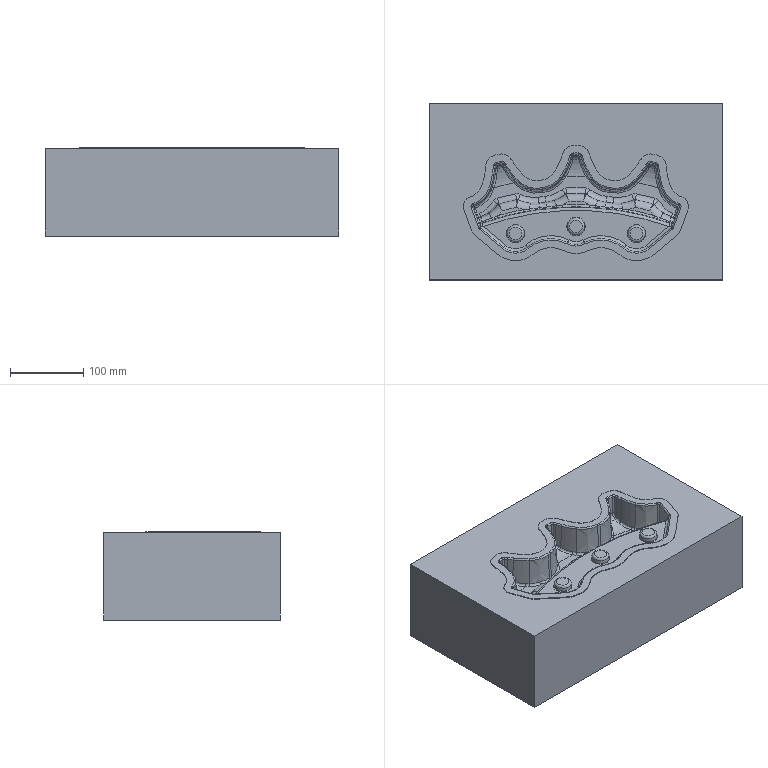CAM job | NX | mm | 3-axis | 1 set-up | 9 operations | part box 400 x 240 x 120
set-up 1
1. Cavity Milling | Mill Mill5 D50R5 | CAVITY_MILL | path 7742.906 mm | 3.09 min
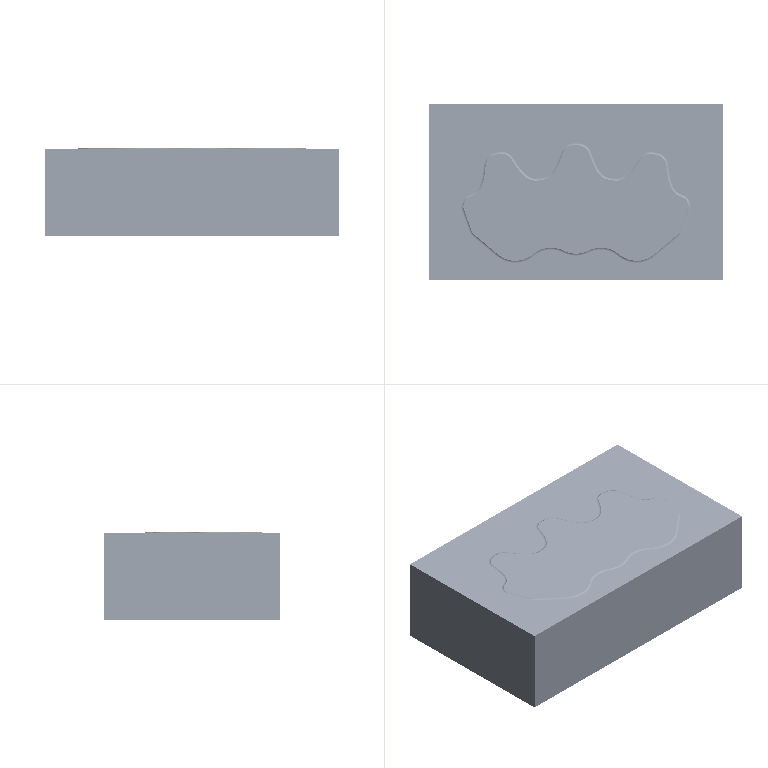2. Cavity Milling | Mill Mill5 D25R5 | CAVITY_MILL_COPY | path 81263.729 mm | 31.134 min
3. Cavity Milling | Mill Mill5 D8 | CAVITY_MILL_COPY_COPY | path 122769.546 mm | 32.411 min
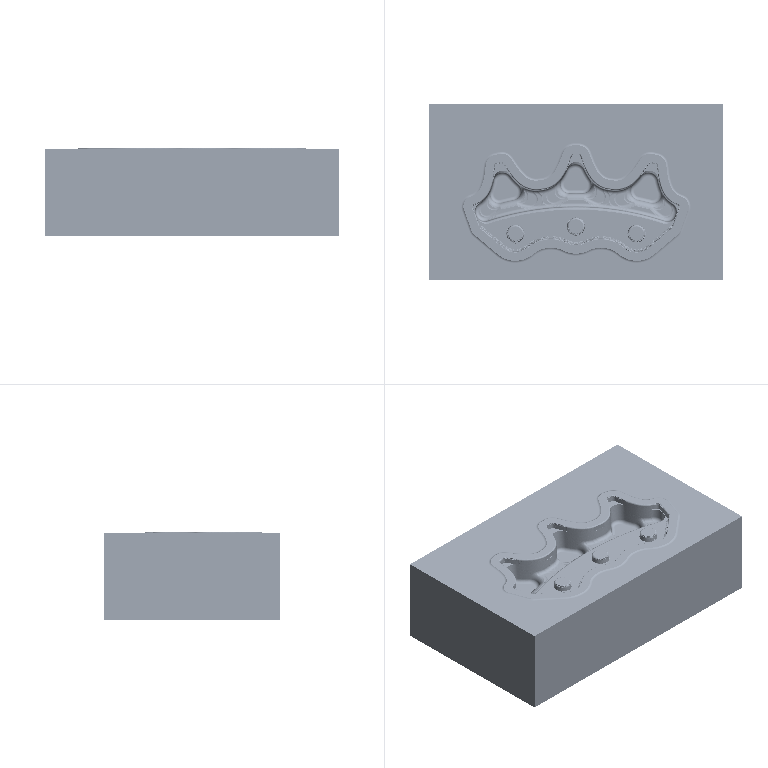4. Z-Level Milling | Mill Mill5 D8 | ZLEVEL_PROFILE | path 58058.454 mm | 23.038 min
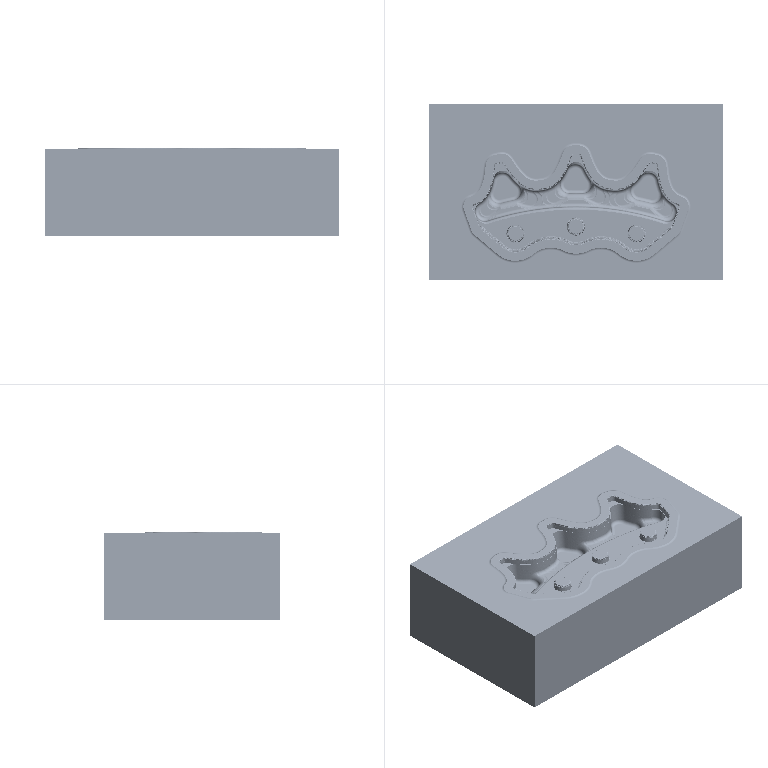5. Face Milling | Mill Mill5 D10 | FACE_MILLING | path 1164.351 mm | 0.455 min
6. Cavity Milling | Mill Mill5 D12 | CAVITY_MILL_COPY_COPY_COPY | path 248708.448 mm | 98.224 min
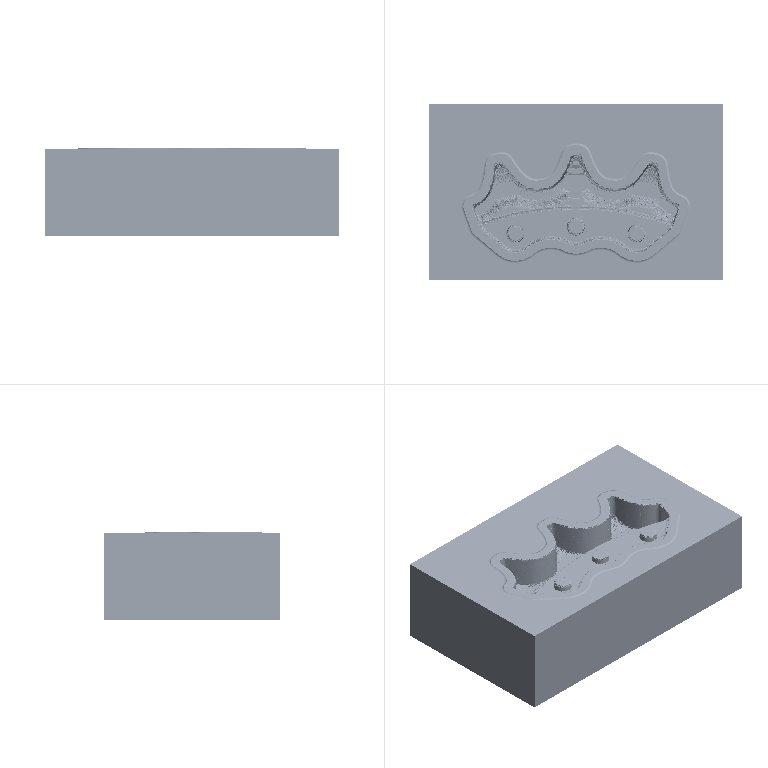7. Face Milling | Mill Mill5 D8R1 | FACE_MILLING_1 | path 2015.213 mm | 0.7953 min
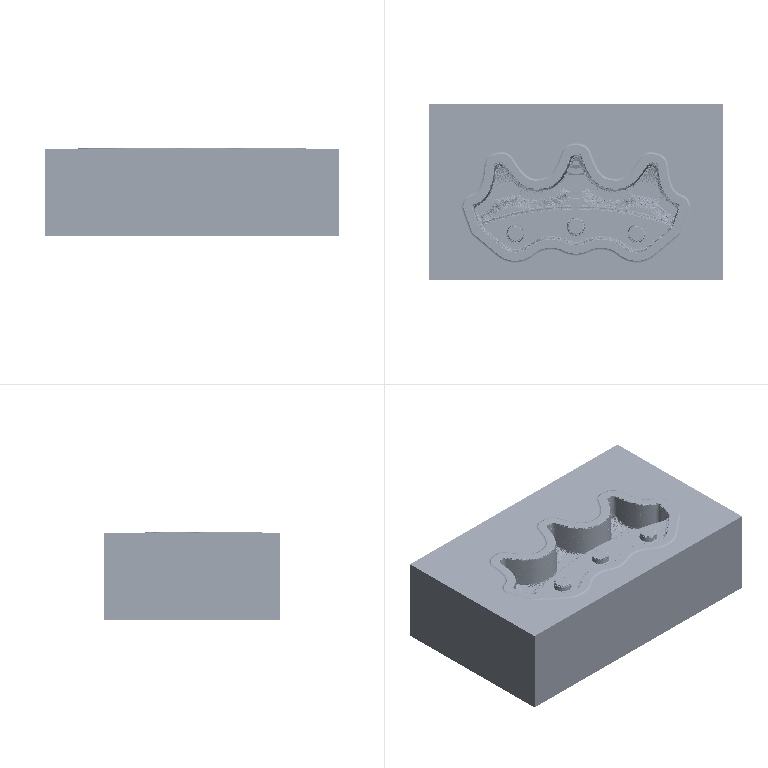8. Z-Level Milling | Mill Mill5 D8R1 | ZLEVEL_PROFILE_COPY | path 222652.808 mm | 88.906 min
9. Fixed-axis Surface Contouring | Mill Mill5 D8R1 | CONTOUR_AREA | path 28664.95 mm | 11.366 min